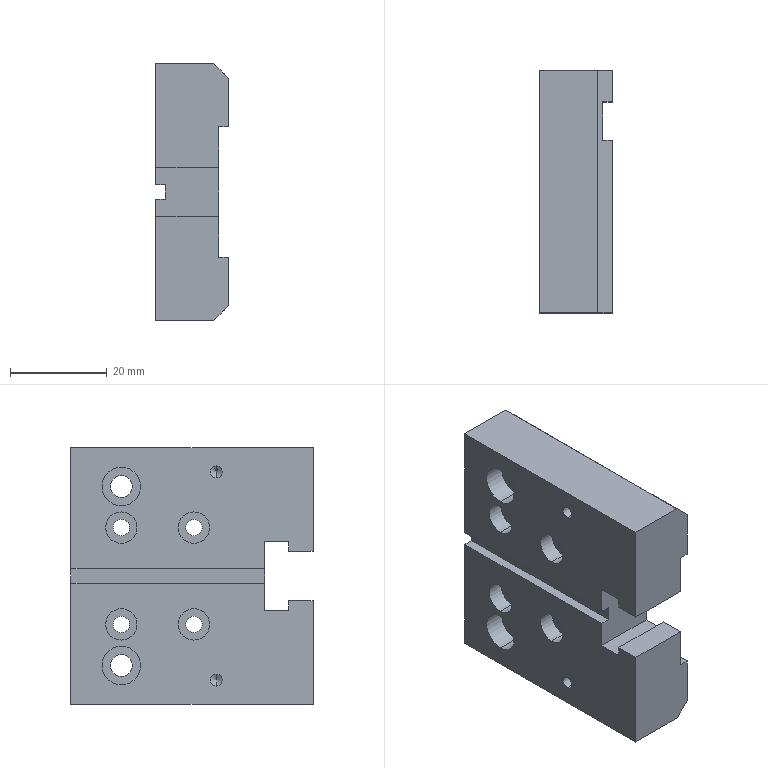Component | SolidWorks | 7.1.02.0001.00.00-0081-1 | 1 solid | 78 faces | box 15 x 50 x 53 mm | volume 32652 mm3 | plane 38 | cylinder 32 | cone 8 | commonest cylinder face diameters 6.5 x8 3.4 x8 2.5 x4 3.3 x4 8 x4 4.5 x4
build123d program:
from build123d import *

# Parameters (mm, degrees)
BOSS_EXTRUDE1_DEPTH                             = 15
M4_HEX_SOCKET_HEAD_CAP_SCREW_CBORE1_D           = 4.5
M4_HEX_SOCKET_HEAD_CAP_SCREW_CBORE1_CBORE_D     = 8
M4_HEX_SOCKET_HEAD_CAP_SCREW_CBORE1_CBORE_DEPTH = 4.4
M3_HEX_SOCKET_HEAD_CAP_SCREW_CBORE1_D           = 3.4
M3_HEX_SOCKET_HEAD_CAP_SCREW_CBORE1_CBORE_D     = 6.5
M3_HEX_SOCKET_HEAD_CAP_SCREW_CBORE1_CBORE_DEPTH = 3.4
SKETCH4_W                                       = 27
SKETCH4_H                                       = 2
CUT_EXTRUDE1_DEPTH                              = 59.543
SKETCH5_W                                       = 2
SKETCH5_H                                       = 8
CUT_EXTRUDE2_DEPTH                              = 61.49
CHAMFER1_SIZE                                   = 3
M4X0_7_TAPPED_HOLE1_D                           = 3.3
M4X0_7_TAPPED_HOLE1_DEPTH                       = 10.1
M4X0_7_TAPPED_HOLE1_TIP                         = 0.9914
M3X0_5_TAPPED_HOLE1_D                           = 2.5
M3X0_5_TAPPED_HOLE1_DEPTH                       = 7.5
M3X0_5_TAPPED_HOLE1_TIP                         = 0.7511
SKETCH9_W                                       = 3
SKETCH9_H                                       = 50
CUT_EXTRUDE3_DEPTH                              = 2


with BuildPart() as part:
    # Sketch1 → Boss-Extrude1 (new body)
    with BuildSketch(Plane.XY):
        Polygon((-5.1, 25), (-5.1, 20), (-7.1, 20), (-7.1, 15), (7.1, 15), (7.1, 20), (5.1, 20), (5.1, 25), (26.5, 25), (26.5, -25), (-26.5, -25), (-26.5, 25), align=None)
    extrude(amount=BOSS_EXTRUDE1_DEPTH)

    # M4 Hex Socket Head Cap Screw CBORE1 (through all)
    with Locations(Plane(origin=(-18.5, -14.6, 15), x_dir=(1, 0, 0), z_dir=(0, 0, 1))):
        with Locations((0, 0), (37, 0)):
            CounterBoreHole(M4_HEX_SOCKET_HEAD_CAP_SCREW_CBORE1_D / 2, M4_HEX_SOCKET_HEAD_CAP_SCREW_CBORE1_CBORE_D / 2, M4_HEX_SOCKET_HEAD_CAP_SCREW_CBORE1_CBORE_DEPTH)

    # M3 Hex Socket Head Cap Screw CBORE1 (through all)
    with Locations(Plane(origin=(-10, 0.4, 15), x_dir=(1, 0, 0), z_dir=(0, 0, 1))):
        with Locations((0, 0), (0, -15), (20, -15), (20, 0)):
            CounterBoreHole(M3_HEX_SOCKET_HEAD_CAP_SCREW_CBORE1_D / 2, M3_HEX_SOCKET_HEAD_CAP_SCREW_CBORE1_CBORE_D / 2, M3_HEX_SOCKET_HEAD_CAP_SCREW_CBORE1_CBORE_DEPTH)

    # Sketch4 → Cut-Extrude1 (cut, through all)
    with BuildSketch(Plane(origin=(0, -25, 0), x_dir=(-1, 0, 0), z_dir=(0, -1, 0))):
        with Locations((0, -1)):
            Rectangle(SKETCH4_W, SKETCH4_H)
    extrude(amount=-CUT_EXTRUDE1_DEPTH, mode=Mode.SUBTRACT)

    # Sketch5 → Cut-Extrude2 (cut, through all)
    with BuildSketch(Plane(origin=(26.5, 0, 0), x_dir=(0, 0, -1), z_dir=(1, 0, 0))):
        with Locations((-1, -14.6)):
            Rectangle(SKETCH5_W, SKETCH5_H)
    extrude(amount=-CUT_EXTRUDE2_DEPTH, mode=Mode.SUBTRACT)

    # Chamfer1
    chamfer1_edges = [part.edges().sort_by_distance(p)[0] for p in [
        (26.5, -21.8, 0),
        (-26.5, -21.8, 0),
    ]]
    chamfer(chamfer1_edges, length=CHAMFER1_SIZE)

    # M4x0.7 Tapped Hole1
    with Locations(Plane(origin=(-4, -25, 8.5), x_dir=(0, 0, -1), z_dir=(0, -1, 0))):
        with Locations((0, 0), (0, 8)):
            Hole(M4X0_7_TAPPED_HOLE1_D / 2, depth=M4X0_7_TAPPED_HOLE1_DEPTH)
            with Locations((0, 0, -(M4X0_7_TAPPED_HOLE1_DEPTH + M4X0_7_TAPPED_HOLE1_TIP / 2))):  # 118° drill point
                Cone(0, M4X0_7_TAPPED_HOLE1_D / 2, M4X0_7_TAPPED_HOLE1_TIP, mode=Mode.SUBTRACT)

    # M3x0.5 Tapped Hole1
    with Locations(Plane(origin=(-21.5, 5, 15), x_dir=(1, 0, 0), z_dir=(0, 0, 1))):
        with Locations((0, 0), (43, 0)):
            Hole(M3X0_5_TAPPED_HOLE1_D / 2, depth=M3X0_5_TAPPED_HOLE1_DEPTH)
            with Locations((0, 0, -(M3X0_5_TAPPED_HOLE1_DEPTH + M3X0_5_TAPPED_HOLE1_TIP / 2))):  # 118° drill point
                Cone(0, M3X0_5_TAPPED_HOLE1_D / 2, M3X0_5_TAPPED_HOLE1_TIP, mode=Mode.SUBTRACT)

    # Sketch9 → Cut-Extrude3 (cut)
    with BuildSketch(Plane.XY.offset(15)):
        Rectangle(SKETCH9_W, SKETCH9_H)
    extrude(amount=-CUT_EXTRUDE3_DEPTH, mode=Mode.SUBTRACT)


solid = part.part

# Placed as in the assembly
solid = solid.moved(Location((-45.964, 18.316, 0), (180, -90, 0)))